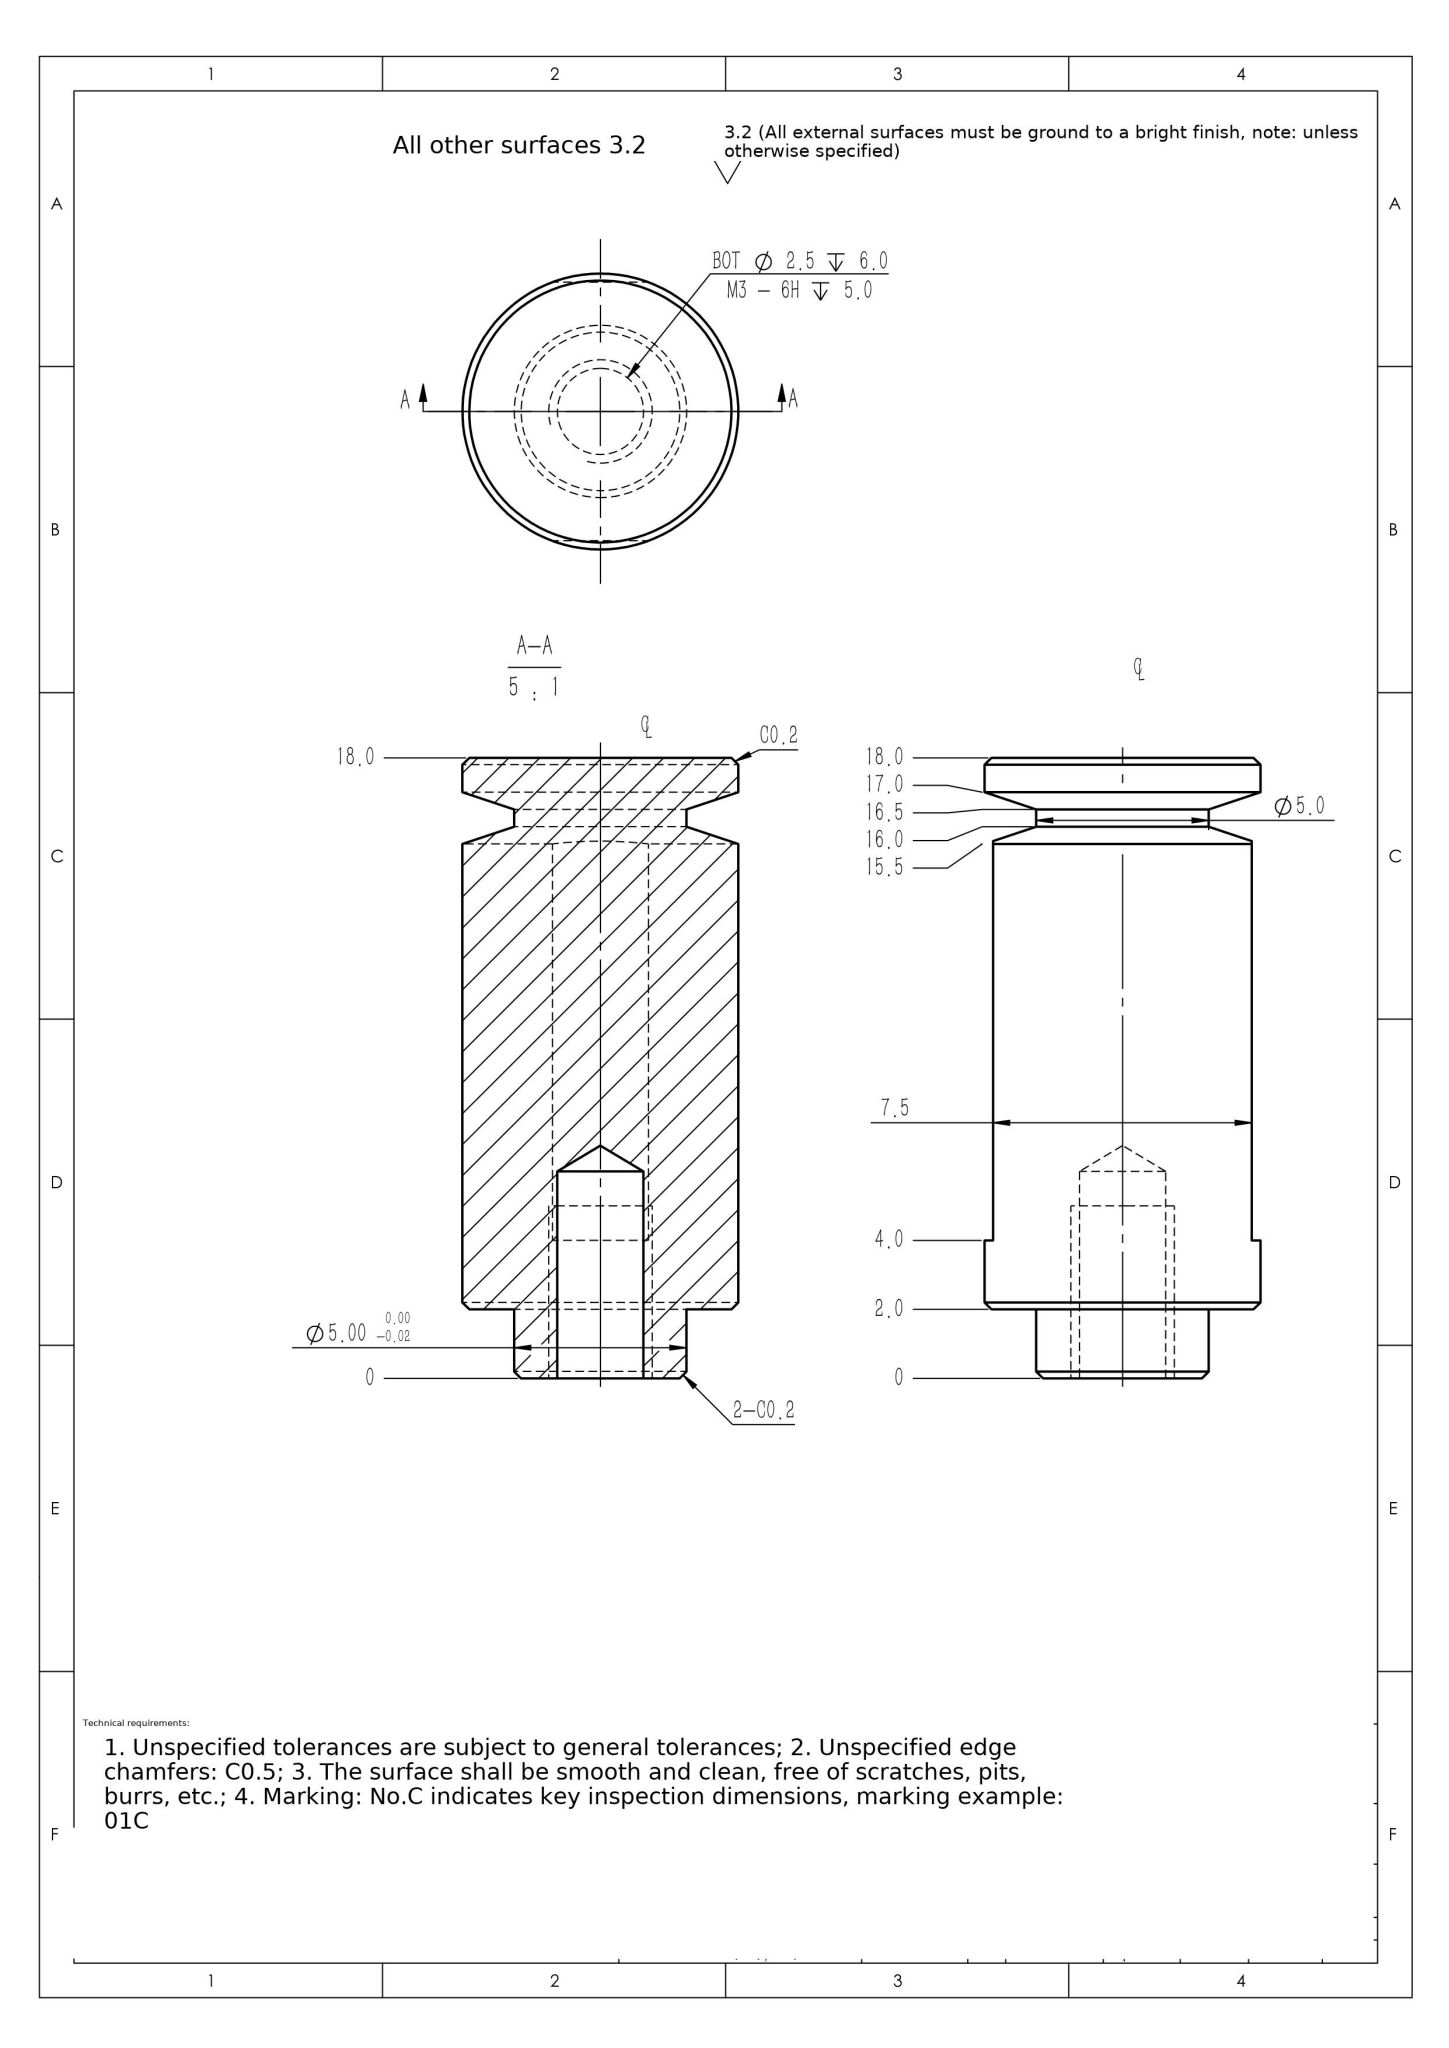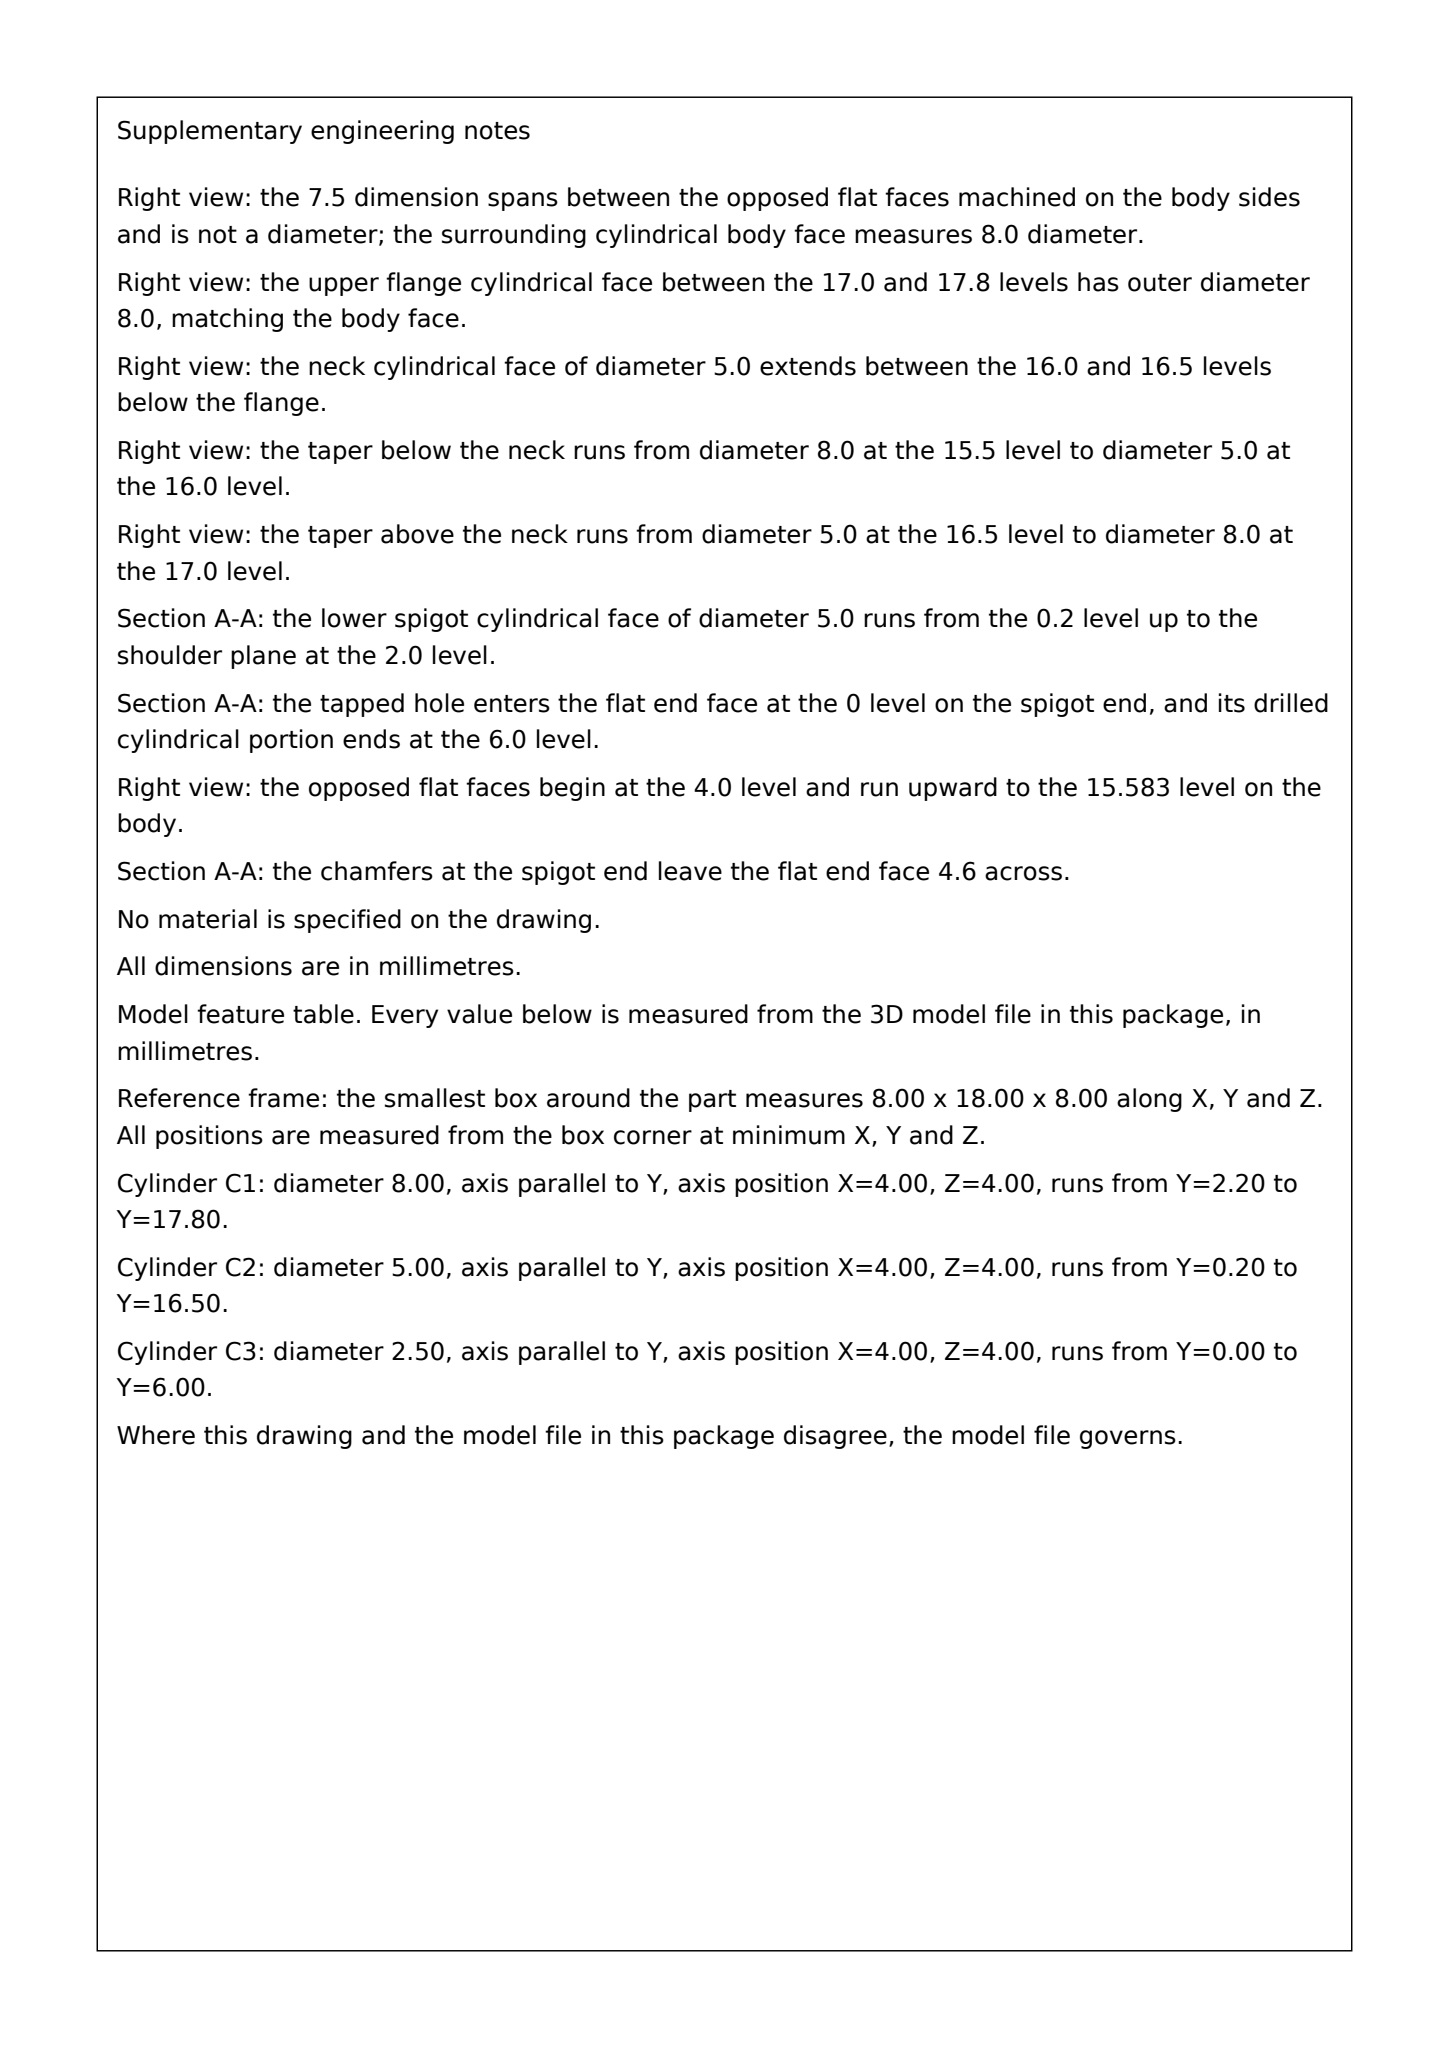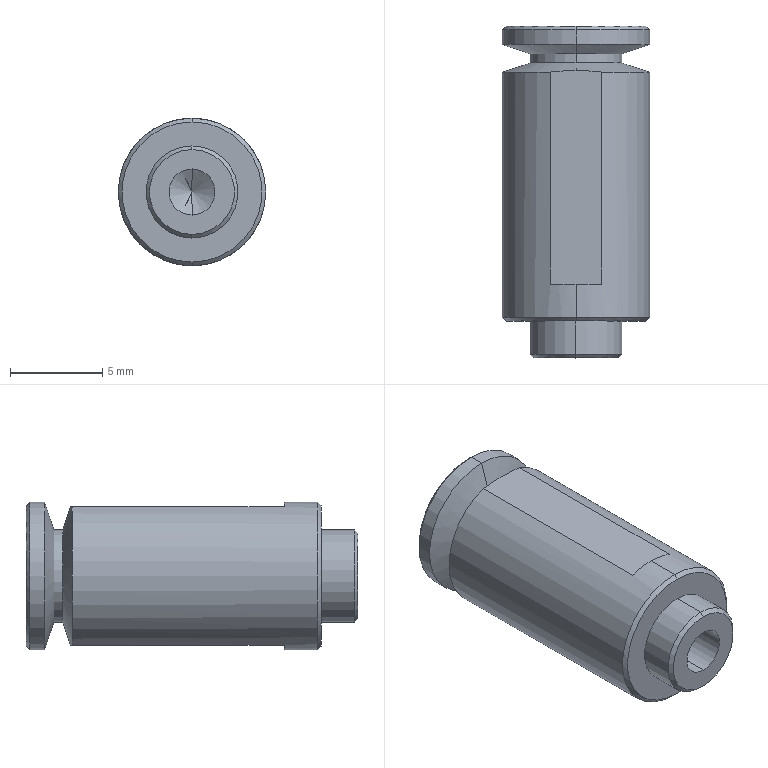Part | SolidWorks | mm | 1 solid | 29 faces | box 8 x 18 x 8 mm | volume 769 mm3 | cone 12 | cylinder 10 | plane 7 | commonest cylinder face diameters 5 x4 8 x4 2.5 x2
Drawing notes:
Ø8.0 BODY & HEAD OD (TYP, SEC A-A) | from the solid: cylinders dia 8.0, axis y, lengths 13.3 and 0.8, pos (4.0,4.0)
C0.2 AT Ø8.0 TO Ø5.00 BOSS SHOULDER, 2.0 FROM BOTTOM | from the solid: axis plane y=2.0 step from Ø8.0 body to Ø5.0 boss; chamfer ref dia 8.0 / 5.0
build123d program:
from build123d import *

# Parameters (mm, degrees)
SKETCH1_R             = 4
BOSS_EXTRUDE1_DEPTH   = 18
M3_TAPPED_HOLE1_D     = 2.5
M3_TAPPED_HOLE1_DEPTH = 6
M3_TAPPED_HOLE1_TIP   = 0.7511
CHAMFER1_SIZE         = 0.2
SKETCH6_W             = 1.126
SKETCH6_H             = 12
SKETCH6_W_2           = 1.355
CUT_EXTRUDE1_DEPTH    = 5
SKETCH9_R             = 4
SKETCH9_R_2           = 2.5
CUT_EXTRUDE2_DEPTH    = 2
CHAMFER2_SIZE         = 0.2


with BuildPart() as part:
    # Sketch1 → Boss-Extrude1 (new body)
    with BuildSketch(Plane(origin=(0, 0, 0), x_dir=(1, 0, 0), z_dir=(0, 1, 0))):
        with Locations(Location((0, 0, 0), (0, 0, 270))):
            Circle(SKETCH1_R)
    extrude(amount=BOSS_EXTRUDE1_DEPTH)

    # M3 Tapped Hole1
    with Locations(Plane(origin=(0, 0, 0), x_dir=(-1, 0, 0), z_dir=(0, -1, 0))):
        with Locations((0, 0)):
            Hole(M3_TAPPED_HOLE1_D / 2, depth=M3_TAPPED_HOLE1_DEPTH)
            with Locations((0, 0, -(M3_TAPPED_HOLE1_DEPTH + M3_TAPPED_HOLE1_TIP / 2))):  # 118° drill point
                Cone(0, M3_TAPPED_HOLE1_D / 2, M3_TAPPED_HOLE1_TIP, mode=Mode.SUBTRACT)

    # Chamfer1
    chamfer1_edges = [part.edges().sort_by_distance(p)[0] for p in [
        (0, 18, -4),
    ]]
    chamfer(chamfer1_edges, length=CHAMFER1_SIZE)

    # Sketch6 → Cut-Extrude1 (cut, symmetric)
    with BuildSketch(Plane(origin=(0, 0, 0), x_dir=(0, 0, -1), z_dir=(1, 0, 0))):
        with Locations((-4.313, 10)):
            Rectangle(SKETCH6_W, SKETCH6_H)
        with Locations((4.427, 10)):
            Rectangle(SKETCH6_W_2, SKETCH6_H)
    extrude(amount=CUT_EXTRUDE1_DEPTH, both=True, mode=Mode.SUBTRACT)

    # Sketch8 → Cut-Revolve1 (revolve, cut)
    with BuildSketch(Plane.XY, mode=Mode.PRIVATE) as cut_revolve1_sk:
        Polygon((-4, 17), (-2.5, 16.5), (-2.5, 16), (-4, 15.5), align=None)
    revolve(cut_revolve1_sk.sketch.rotate(Axis((0, 18, 0), (0, -1, 0)), 69.636), axis=Axis((0, 18, 0), (0, -1, 0)), mode=Mode.SUBTRACT)

    # Sketch9 → Cut-Extrude2 (cut)
    with BuildSketch(Plane.XZ):
        with Locations(Location((0, 0, 0), (0, 0, 270))):
            Circle(SKETCH9_R)
        with Locations(Location((0, 0, 0), (0, 0, 90))):
            Circle(SKETCH9_R_2, mode=Mode.SUBTRACT)
    extrude(amount=-CUT_EXTRUDE2_DEPTH, mode=Mode.SUBTRACT)

    # Chamfer2
    chamfer2_edges = [part.edges().sort_by_distance(p)[0] for p in [
        (0, 2, -4),
        (0, 0, -2.5),
    ]]
    chamfer(chamfer2_edges, length=CHAMFER2_SIZE)


solid = part.part
STEP:
#1=CARTESIAN_POINT('',(-0.,0.,-2.3));
#2=VERTEX_POINT('',#1);
#3=CARTESIAN_POINT('',(-0.,0.,2.3));
#4=VERTEX_POINT('',#3);
#5=CARTESIAN_POINT('',(-0.,0.,0.));
#6=DIRECTION('',(0.,-1.,0.));
#7=DIRECTION('',(0.,0.,1.));
#8=AXIS2_PLACEMENT_3D('',#5,#6,#7);
#9=CIRCLE('',#8,2.3);
#10=EDGE_CURVE('',#2,#4,#9,.T.);
#11=ORIENTED_EDGE('',*,*,#10,.F.);
#12=CARTESIAN_POINT('',(-0.,0.2,-2.5));
#13=VERTEX_POINT('',#12);
#14=CARTESIAN_POINT('',(-0.,0.,-2.3));
#15=DIRECTION('',(0.,0.7071,-0.7071));
#16=VECTOR('',#15,1000.);
#17=LINE('',#14,#16);
#18=EDGE_CURVE('',#2,#13,#17,.T.);
#19=ORIENTED_EDGE('',*,*,#18,.T.);
#20=CARTESIAN_POINT('',(-0.,0.2,2.5));
#21=VERTEX_POINT('',#20);
#22=CARTESIAN_POINT('',(-0.,0.2,0.));
#23=DIRECTION('',(0.,1.,0.));
#24=DIRECTION('',(0.,0.,1.));
#25=AXIS2_PLACEMENT_3D('',#22,#23,#24);
#26=CIRCLE('',#25,2.5);
#27=EDGE_CURVE('',#21,#13,#26,.T.);
#28=ORIENTED_EDGE('',*,*,#27,.F.);
#29=CARTESIAN_POINT('',(-0.,0.,2.3));
#30=DIRECTION('',(0.,0.7071,0.7071));
#31=VECTOR('',#30,1000.);
#32=LINE('',#29,#31);
#33=EDGE_CURVE('',#4,#21,#32,.T.);
#34=ORIENTED_EDGE('',*,*,#33,.F.);
#35=EDGE_LOOP('',(#11,#19,#28,#34));
#36=FACE_OUTER_BOUND('',#35,.T.);
#37=CARTESIAN_POINT('',(-0.,0.,0.));
#38=DIRECTION('',(0.,1.,0.));
#39=DIRECTION('',(0.,0.,1.));
#40=AXIS2_PLACEMENT_3D('',#37,#38,#39);
#41=CONICAL_SURFACE('',#40,2.3,0.7854);
#42=ADVANCED_FACE('',(#36),#41,.T.);
#43=CARTESIAN_POINT('',(0.,2.,-3.8));
#44=VERTEX_POINT('',#43);
#45=CARTESIAN_POINT('',(0.,2.,3.8));
#46=VERTEX_POINT('',#45);
#47=CARTESIAN_POINT('',(0.,2.,0.));
#48=DIRECTION('',(0.,-1.,0.));
#49=DIRECTION('',(0.,0.,-1.));
#50=AXIS2_PLACEMENT_3D('',#47,#48,#49);
#51=CIRCLE('',#50,3.8);
#52=EDGE_CURVE('',#44,#46,#51,.T.);
#53=ORIENTED_EDGE('',*,*,#52,.F.);
#54=CARTESIAN_POINT('',(0.,2.2,-4.));
#55=VERTEX_POINT('',#54);
#56=CARTESIAN_POINT('',(0.,2.,-3.8));
#57=DIRECTION('',(0.,0.7071,-0.7071));
#58=VECTOR('',#57,1000.);
#59=LINE('',#56,#58);
#60=EDGE_CURVE('',#44,#55,#59,.T.);
#61=ORIENTED_EDGE('',*,*,#60,.T.);
#62=CARTESIAN_POINT('',(0.,2.2,4.));
#63=VERTEX_POINT('',#62);
#64=CARTESIAN_POINT('',(0.,2.2,0.));
#65=DIRECTION('',(0.,1.,0.));
#66=DIRECTION('',(0.,0.,-1.));
#67=AXIS2_PLACEMENT_3D('',#64,#65,#66);
#68=CIRCLE('',#67,4.);
#69=EDGE_CURVE('',#63,#55,#68,.T.);
#70=ORIENTED_EDGE('',*,*,#69,.F.);
#71=CARTESIAN_POINT('',(0.,2.,3.8));
#72=DIRECTION('',(0.,0.7071,0.7071));
#73=VECTOR('',#72,1000.);
#74=LINE('',#71,#73);
#75=EDGE_CURVE('',#46,#63,#74,.T.);
#76=ORIENTED_EDGE('',*,*,#75,.F.);
#77=EDGE_LOOP('',(#53,#61,#70,#76));
#78=FACE_OUTER_BOUND('',#77,.T.);
#79=CARTESIAN_POINT('',(0.,2.,0.));
#80=DIRECTION('',(0.,1.,0.));
#81=DIRECTION('',(0.,0.,1.));
#82=AXIS2_PLACEMENT_3D('',#79,#80,#81);
#83=CONICAL_SURFACE('',#82,3.8,0.7854);
#84=ADVANCED_FACE('',(#78),#83,.T.);
#85=CARTESIAN_POINT('',(0.,6.,1.25));
#86=VERTEX_POINT('',#85);
#87=CARTESIAN_POINT('',(0.,6.,-1.25));
#88=VERTEX_POINT('',#87);
#89=CARTESIAN_POINT('',(0.,6.,0.));
#90=DIRECTION('',(0.,-1.,0.));
#91=DIRECTION('',(0.,0.,-1.));
#92=AXIS2_PLACEMENT_3D('',#89,#90,#91);
#93=CIRCLE('',#92,1.25);
#94=EDGE_CURVE('',#86,#88,#93,.T.);
#95=ORIENTED_EDGE('',*,*,#94,.F.);
#96=CARTESIAN_POINT('',(0.,-0.,1.25));
#97=VERTEX_POINT('',#96);
#98=CARTESIAN_POINT('',(0.,0.,1.25));
#99=DIRECTION('',(0.,-1.,0.));
#100=VECTOR('',#99,1000.);
#101=LINE('',#98,#100);
#102=EDGE_CURVE('',#86,#97,#101,.T.);
#103=ORIENTED_EDGE('',*,*,#102,.T.);
#104=CARTESIAN_POINT('',(0.,-0.,-1.25));
#105=VERTEX_POINT('',#104);
#106=CARTESIAN_POINT('',(0.,-0.,0.));
#107=DIRECTION('',(0.,-1.,0.));
#108=DIRECTION('',(0.,0.,-1.));
#109=AXIS2_PLACEMENT_3D('',#106,#107,#108);
#110=CIRCLE('',#109,1.25);
#111=EDGE_CURVE('',#97,#105,#110,.T.);
#112=ORIENTED_EDGE('',*,*,#111,.T.);
#113=CARTESIAN_POINT('',(0.,0.,-1.25));
#114=DIRECTION('',(0.,-1.,0.));
#115=VECTOR('',#114,1000.);
#116=LINE('',#113,#115);
#117=EDGE_CURVE('',#88,#105,#116,.T.);
#118=ORIENTED_EDGE('',*,*,#117,.F.);
#119=EDGE_LOOP('',(#95,#103,#112,#118));
#120=FACE_OUTER_BOUND('',#119,.T.);
#121=CARTESIAN_POINT('',(0.,0.,0.));
#122=DIRECTION('',(0.,-1.,0.));
#123=DIRECTION('',(0.,0.,-1.));
#124=AXIS2_PLACEMENT_3D('',#121,#122,#123);
#125=CYLINDRICAL_SURFACE('',#124,1.25);
#126=ADVANCED_FACE('',(#120),#125,.F.);
#127=CARTESIAN_POINT('',(-0.,6.751,0.));
#128=VERTEX_POINT('',#127);
#129=CARTESIAN_POINT('',(0.,6.,-1.25));
#130=DIRECTION('',(0.,-0.515,-0.8572));
#131=VECTOR('',#130,1000.);
#132=LINE('',#129,#131);
#133=EDGE_CURVE('',#128,#88,#132,.T.);
#134=ORIENTED_EDGE('',*,*,#133,.F.);
#135=CARTESIAN_POINT('',(0.,6.,1.25));
#136=DIRECTION('',(0.,-0.515,0.8572));
#137=VECTOR('',#136,1000.);
#138=LINE('',#135,#137);
#139=EDGE_CURVE('',#128,#86,#138,.T.);
#140=ORIENTED_EDGE('',*,*,#139,.T.);
#141=ORIENTED_EDGE('',*,*,#94,.T.);
#142=EDGE_LOOP('',(#134,#140,#141));
#143=FACE_OUTER_BOUND('',#142,.T.);
#144=CARTESIAN_POINT('',(0.,6.,0.));
#145=DIRECTION('',(0.,-1.,0.));
#146=DIRECTION('',(0.,0.,-1.));
#147=AXIS2_PLACEMENT_3D('',#144,#145,#146);
#148=CONICAL_SURFACE('',#147,1.25,1.03);
#149=ADVANCED_FACE('',(#143),#148,.F.);
#150=CARTESIAN_POINT('',(-0.,2.,-2.5));
#151=VERTEX_POINT('',#150);
#152=CARTESIAN_POINT('',(-0.,2.,2.5));
#153=VERTEX_POINT('',#152);
#154=CARTESIAN_POINT('',(-0.,2.,0.));
#155=DIRECTION('',(0.,-1.,0.));
#156=DIRECTION('',(0.,0.,-1.));
#157=AXIS2_PLACEMENT_3D('',#154,#155,#156);
#158=CIRCLE('',#157,2.5);
#159=EDGE_CURVE('',#151,#153,#158,.T.);
#160=ORIENTED_EDGE('',*,*,#159,.T.);
#161=CARTESIAN_POINT('',(-0.,2.,2.5));
#162=DIRECTION('',(0.,-1.,0.));
#163=VECTOR('',#162,1000.);
#164=LINE('',#161,#163);
#165=EDGE_CURVE('',#153,#21,#164,.T.);
#166=ORIENTED_EDGE('',*,*,#165,.T.);
#167=ORIENTED_EDGE('',*,*,#27,.T.);
#168=CARTESIAN_POINT('',(-0.,2.,-2.5));
#169=DIRECTION('',(0.,-1.,0.));
#170=VECTOR('',#169,1000.);
#171=LINE('',#168,#170);
#172=EDGE_CURVE('',#151,#13,#171,.T.);
#173=ORIENTED_EDGE('',*,*,#172,.F.);
#174=EDGE_LOOP('',(#160,#166,#167,#173));
#175=FACE_OUTER_BOUND('',#174,.T.);
#176=CARTESIAN_POINT('',(-0.,2.,0.));
#177=DIRECTION('',(0.,-1.,0.));
#178=DIRECTION('',(0.,0.,-1.));
#179=AXIS2_PLACEMENT_3D('',#176,#177,#178);
#180=CYLINDRICAL_SURFACE('',#179,2.5);
#181=ADVANCED_FACE('',(#175),#180,.T.);
#182=CARTESIAN_POINT('',(0.,17.8,-4.));
#183=VERTEX_POINT('',#182);
#184=CARTESIAN_POINT('',(0.,17.8,4.));
#185=VERTEX_POINT('',#184);
#186=CARTESIAN_POINT('',(0.,17.8,0.));
#187=DIRECTION('',(0.,-1.,0.));
#188=DIRECTION('',(0.,0.,1.));
#189=AXIS2_PLACEMENT_3D('',#186,#187,#188);
#190=CIRCLE('',#189,4.);
#191=EDGE_CURVE('',#183,#185,#190,.T.);
#192=ORIENTED_EDGE('',*,*,#191,.T.);
#193=CARTESIAN_POINT('',(0.,17.,4.));
#194=VERTEX_POINT('',#193);
#195=CARTESIAN_POINT('',(0.,18.,4.));
#196=DIRECTION('',(0.,-1.,0.));
#197=VECTOR('',#196,1000.);
#198=LINE('',#195,#197);
#199=EDGE_CURVE('',#185,#194,#198,.T.);
#200=ORIENTED_EDGE('',*,*,#199,.T.);
#201=CARTESIAN_POINT('',(0.,17.,-4.));
#202=VERTEX_POINT('',#201);
#203=CARTESIAN_POINT('',(0.,17.,0.));
#204=DIRECTION('',(0.,1.,0.));
#205=DIRECTION('',(0.,0.,1.));
#206=AXIS2_PLACEMENT_3D('',#203,#204,#205);
#207=CIRCLE('',#206,4.);
#208=EDGE_CURVE('',#194,#202,#207,.T.);
#209=ORIENTED_EDGE('',*,*,#208,.T.);
#210=CARTESIAN_POINT('',(0.,18.,-4.));
#211=DIRECTION('',(0.,-1.,0.));
#212=VECTOR('',#211,1000.);
#213=LINE('',#210,#212);
#214=EDGE_CURVE('',#183,#202,#213,.T.);
#215=ORIENTED_EDGE('',*,*,#214,.F.);
#216=EDGE_LOOP('',(#192,#200,#209,#215));
#217=FACE_OUTER_BOUND('',#216,.T.);
#218=CARTESIAN_POINT('',(0.,18.,0.));
#219=DIRECTION('',(0.,-1.,0.));
#220=DIRECTION('',(0.,0.,-1.));
#221=AXIS2_PLACEMENT_3D('',#218,#219,#220);
#222=CYLINDRICAL_SURFACE('',#221,4.);
#223=ADVANCED_FACE('',(#217),#222,.T.);
#224=CARTESIAN_POINT('',(0.,18.,3.8));
#225=VERTEX_POINT('',#224);
#226=CARTESIAN_POINT('',(0.,18.,-3.8));
#227=VERTEX_POINT('',#226);
#228=CARTESIAN_POINT('',(0.,18.,0.));
#229=DIRECTION('',(0.,1.,0.));
#230=DIRECTION('',(0.,0.,1.));
#231=AXIS2_PLACEMENT_3D('',#228,#229,#230);
#232=CIRCLE('',#231,3.8);
#233=EDGE_CURVE('',#225,#227,#232,.T.);
#234=ORIENTED_EDGE('',*,*,#233,.F.);
#235=CARTESIAN_POINT('',(0.,18.,3.8));
#236=DIRECTION('',(0.,-0.7071,0.7071));
#237=VECTOR('',#236,1000.);
#238=LINE('',#235,#237);
#239=EDGE_CURVE('',#225,#185,#238,.T.);
#240=ORIENTED_EDGE('',*,*,#239,.T.);
#241=ORIENTED_EDGE('',*,*,#191,.F.);
#242=CARTESIAN_POINT('',(0.,18.,-3.8));
#243=DIRECTION('',(0.,-0.7071,-0.7071));
#244=VECTOR('',#243,1000.);
#245=LINE('',#242,#244);
#246=EDGE_CURVE('',#227,#183,#245,.T.);
#247=ORIENTED_EDGE('',*,*,#246,.F.);
#248=EDGE_LOOP('',(#234,#240,#241,#247));
#249=FACE_OUTER_BOUND('',#248,.T.);
#250=CARTESIAN_POINT('',(0.,18.,0.));
#251=DIRECTION('',(0.,-1.,0.));
#252=DIRECTION('',(0.,0.,-1.));
#253=AXIS2_PLACEMENT_3D('',#250,#251,#252);
#254=CONICAL_SURFACE('',#253,3.8,0.7854);
#255=ADVANCED_FACE('',(#249),#254,.T.);
#256=CARTESIAN_POINT('',(0.,16.,2.5));
#257=VERTEX_POINT('',#256);
#258=CARTESIAN_POINT('',(0.,16.,-2.5));
#259=VERTEX_POINT('',#258);
#260=CARTESIAN_POINT('',(0.,16.,0.));
#261=DIRECTION('',(0.,1.,0.));
#262=DIRECTION('',(0.,0.,1.));
#263=AXIS2_PLACEMENT_3D('',#260,#261,#262);
#264=CIRCLE('',#263,2.5);
#265=EDGE_CURVE('',#257,#259,#264,.T.);
#266=ORIENTED_EDGE('',*,*,#265,.T.);
#267=CARTESIAN_POINT('',(0.,16.5,-2.5));
#268=VERTEX_POINT('',#267);
#269=CARTESIAN_POINT('',(0.,18.,-2.5));
#270=DIRECTION('',(0.,1.,0.));
#271=VECTOR('',#270,1000.);
#272=LINE('',#269,#271);
#273=EDGE_CURVE('',#259,#268,#272,.T.);
#274=ORIENTED_EDGE('',*,*,#273,.T.);
#275=CARTESIAN_POINT('',(0.,16.5,2.5));
#276=VERTEX_POINT('',#275);
#277=CARTESIAN_POINT('',(0.,16.5,0.));
#278=DIRECTION('',(0.,1.,0.));
#279=DIRECTION('',(0.,0.,1.));
#280=AXIS2_PLACEMENT_3D('',#277,#278,#279);
#281=CIRCLE('',#280,2.5);
#282=EDGE_CURVE('',#276,#268,#281,.T.);
#283=ORIENTED_EDGE('',*,*,#282,.F.);
#284=CARTESIAN_POINT('',(0.,18.,2.5));
#285=DIRECTION('',(0.,1.,0.));
#286=VECTOR('',#285,1000.);
#287=LINE('',#284,#286);
#288=EDGE_CURVE('',#257,#276,#287,.T.);
#289=ORIENTED_EDGE('',*,*,#288,.F.);
#290=EDGE_LOOP('',(#266,#274,#283,#289));
#291=FACE_OUTER_BOUND('',#290,.T.);
#292=CARTESIAN_POINT('',(0.,18.,0.));
#293=DIRECTION('',(0.,1.,0.));
#294=DIRECTION('',(0.,0.,1.));
#295=AXIS2_PLACEMENT_3D('',#292,#293,#294);
#296=CYLINDRICAL_SURFACE('',#295,2.5);
#297=ADVANCED_FACE('',(#291),#296,.T.);
#298=ORIENTED_EDGE('',*,*,#282,.T.);
#299=CARTESIAN_POINT('',(0.,16.5,-2.5));
#300=DIRECTION('',(0.,0.3162,-0.9487));
#301=VECTOR('',#300,1000.);
#302=LINE('',#299,#301);
#303=EDGE_CURVE('',#268,#202,#302,.T.);
#304=ORIENTED_EDGE('',*,*,#303,.T.);
#305=ORIENTED_EDGE('',*,*,#208,.F.);
#306=CARTESIAN_POINT('',(0.,16.5,2.5));
#307=DIRECTION('',(0.,0.3162,0.9487));
#308=VECTOR('',#307,1000.);
#309=LINE('',#306,#308);
#310=EDGE_CURVE('',#276,#194,#309,.T.);
#311=ORIENTED_EDGE('',*,*,#310,.F.);
#312=EDGE_LOOP('',(#298,#304,#305,#311));
#313=FACE_OUTER_BOUND('',#312,.T.);
#314=CARTESIAN_POINT('',(0.,16.5,0.));
#315=DIRECTION('',(0.,1.,0.));
#316=DIRECTION('',(0.,0.,1.));
#317=AXIS2_PLACEMENT_3D('',#314,#315,#316);
#318=CONICAL_SURFACE('',#317,2.5,1.249);
#319=ADVANCED_FACE('',(#313),#318,.T.);
#320=ORIENTED_EDGE('',*,*,#265,.F.);
#321=CARTESIAN_POINT('',(0.,15.583,3.75));
#322=VERTEX_POINT('',#321);
#323=CARTESIAN_POINT('',(0.,15.5,4.));
#324=DIRECTION('',(0.,-0.3162,0.9487));
#325=VECTOR('',#324,1000.);
#326=LINE('',#323,#325);
#327=EDGE_CURVE('',#257,#322,#326,.T.);
#328=ORIENTED_EDGE('',*,*,#327,.T.);
#329=CARTESIAN_POINT('',(1.392,15.5,3.75));
#330=VERTEX_POINT('',#329);
#331=CARTESIAN_POINT('',(1.392,15.5,3.75));
#332=CARTESIAN_POINT('',(0.9298,15.554,3.75));
#333=CARTESIAN_POINT('',(0.466,15.583,3.75));
#334=CARTESIAN_POINT('',(0.,15.583,3.75));
#335=B_SPLINE_CURVE_WITH_KNOTS('',3,(#331,#332,#333,#334),.UNSPECIFIED.,.F.,.F.,(4,4),(0.001505,0.002899),.UNSPECIFIED.);
#336=EDGE_CURVE('',#330,#322,#335,.T.);
#337=ORIENTED_EDGE('',*,*,#336,.F.);
#338=CARTESIAN_POINT('',(1.392,15.5,-3.75));
#339=VERTEX_POINT('',#338);
#340=CARTESIAN_POINT('',(0.,15.5,0.));
#341=DIRECTION('',(0.,1.,0.));
#342=DIRECTION('',(0.,0.,1.));
#343=AXIS2_PLACEMENT_3D('',#340,#341,#342);
#344=CIRCLE('',#343,4.);
#345=EDGE_CURVE('',#330,#339,#344,.T.);
#346=ORIENTED_EDGE('',*,*,#345,.T.);
#347=CARTESIAN_POINT('',(0.,15.583,-3.75));
#348=VERTEX_POINT('',#347);
#349=CARTESIAN_POINT('',(0.,15.583,-3.75));
#350=CARTESIAN_POINT('',(0.466,15.583,-3.75));
#351=CARTESIAN_POINT('',(0.9298,15.554,-3.75));
#352=CARTESIAN_POINT('',(1.392,15.5,-3.75));
#353=B_SPLINE_CURVE_WITH_KNOTS('',3,(#349,#350,#351,#352),.UNSPECIFIED.,.F.,.F.,(4,4),(0.005039,0.006443),.UNSPECIFIED.);
#354=EDGE_CURVE('',#348,#339,#353,.T.);
#355=ORIENTED_EDGE('',*,*,#354,.F.);
#356=CARTESIAN_POINT('',(0.,15.5,-4.));
#357=DIRECTION('',(0.,-0.3162,-0.9487));
#358=VECTOR('',#357,1000.);
#359=LINE('',#356,#358);
#360=EDGE_CURVE('',#259,#348,#359,.T.);
#361=ORIENTED_EDGE('',*,*,#360,.F.);
#362=EDGE_LOOP('',(#320,#328,#337,#346,#355,#361));
#363=FACE_OUTER_BOUND('',#362,.T.);
#364=CARTESIAN_POINT('',(0.,15.5,0.));
#365=DIRECTION('',(0.,-1.,0.));
#366=DIRECTION('',(0.,0.,-1.));
#367=AXIS2_PLACEMENT_3D('',#364,#365,#366);
#368=CONICAL_SURFACE('',#367,4.,1.249);
#369=ADVANCED_FACE('',(#363),#368,.T.);
#370=CARTESIAN_POINT('',(1.392,4.,3.75));
#371=VERTEX_POINT('',#370);
#372=CARTESIAN_POINT('',(0.,4.,4.));
#373=VERTEX_POINT('',#372);
#374=CARTESIAN_POINT('',(0.,4.,0.));
#375=DIRECTION('',(0.,-1.,0.));
#376=DIRECTION('',(0.,0.,-1.));
#377=AXIS2_PLACEMENT_3D('',#374,#375,#376);
#378=CIRCLE('',#377,4.);
#379=EDGE_CURVE('',#371,#373,#378,.T.);
#380=ORIENTED_EDGE('',*,*,#379,.T.);
#381=CARTESIAN_POINT('',(0.,18.,4.));
#382=DIRECTION('',(0.,-1.,0.));
#383=VECTOR('',#382,1000.);
#384=LINE('',#381,#383);
#385=EDGE_CURVE('',#373,#63,#384,.T.);
#386=ORIENTED_EDGE('',*,*,#385,.T.);
#387=ORIENTED_EDGE('',*,*,#69,.T.);
#388=CARTESIAN_POINT('',(0.,4.,-4.));
#389=VERTEX_POINT('',#388);
#390=CARTESIAN_POINT('',(0.,18.,-4.));
#391=DIRECTION('',(0.,-1.,0.));
#392=VECTOR('',#391,1000.);
#393=LINE('',#390,#392);
#394=EDGE_CURVE('',#389,#55,#393,.T.);
#395=ORIENTED_EDGE('',*,*,#394,.F.);
#396=CARTESIAN_POINT('',(1.392,4.,-3.75));
#397=VERTEX_POINT('',#396);
#398=CARTESIAN_POINT('',(0.,4.,0.));
#399=DIRECTION('',(0.,-1.,0.));
#400=DIRECTION('',(0.,0.,-1.));
#401=AXIS2_PLACEMENT_3D('',#398,#399,#400);
#402=CIRCLE('',#401,4.);
#403=EDGE_CURVE('',#389,#397,#402,.T.);
#404=ORIENTED_EDGE('',*,*,#403,.T.);
#405=CARTESIAN_POINT('',(1.392,18.,-3.75));
#406=DIRECTION('',(0.,1.,0.));
#407=VECTOR('',#406,1000.);
#408=LINE('',#405,#407);
#409=EDGE_CURVE('',#397,#339,#408,.T.);
#410=ORIENTED_EDGE('',*,*,#409,.T.);
#411=ORIENTED_EDGE('',*,*,#345,.F.);
#412=CARTESIAN_POINT('',(1.392,18.,3.75));
#413=DIRECTION('',(0.,-1.,0.));
#414=VECTOR('',#413,1000.);
#415=LINE('',#412,#414);
#416=EDGE_CURVE('',#330,#371,#415,.T.);
#417=ORIENTED_EDGE('',*,*,#416,.T.);
#418=EDGE_LOOP('',(#380,#386,#387,#395,#404,#410,#411,#417));
#419=FACE_OUTER_BOUND('',#418,.T.);
#420=CARTESIAN_POINT('',(0.,18.,0.));
#421=DIRECTION('',(0.,-1.,0.));
#422=DIRECTION('',(0.,0.,-1.));
#423=AXIS2_PLACEMENT_3D('',#420,#421,#422);
#424=CYLINDRICAL_SURFACE('',#423,4.);
#425=ADVANCED_FACE('',(#419),#424,.T.);
#426=ORIENTED_EDGE('',*,*,#385,.F.);
#427=CARTESIAN_POINT('',(-1.392,4.,3.75));
#428=VERTEX_POINT('',#427);
#429=CARTESIAN_POINT('',(0.,4.,0.));
#430=DIRECTION('',(0.,-1.,0.));
#431=DIRECTION('',(0.,0.,-1.));
#432=AXIS2_PLACEMENT_3D('',#429,#430,#431);
#433=CIRCLE('',#432,4.);
#434=EDGE_CURVE('',#373,#428,#433,.T.);
#435=ORIENTED_EDGE('',*,*,#434,.T.);
#436=CARTESIAN_POINT('',(-1.392,15.5,3.75));
#437=VERTEX_POINT('',#436);
#438=CARTESIAN_POINT('',(-1.392,18.,3.75));
#439=DIRECTION('',(0.,1.,0.));
#440=VECTOR('',#439,1000.);
#441=LINE('',#438,#440);
#442=EDGE_CURVE('',#428,#437,#441,.T.);
#443=ORIENTED_EDGE('',*,*,#442,.T.);
#444=CARTESIAN_POINT('',(-1.392,15.5,-3.75));
#445=VERTEX_POINT('',#444);
#446=CARTESIAN_POINT('',(0.,15.5,0.));
#447=DIRECTION('',(0.,1.,0.));
#448=DIRECTION('',(0.,0.,1.));
#449=AXIS2_PLACEMENT_3D('',#446,#447,#448);
#450=CIRCLE('',#449,4.);
#451=EDGE_CURVE('',#445,#437,#450,.T.);
#452=ORIENTED_EDGE('',*,*,#451,.F.);
#453=CARTESIAN_POINT('',(-1.392,4.,-3.75));
#454=VERTEX_POINT('',#453);
#455=CARTESIAN_POINT('',(-1.392,18.,-3.75));
#456=DIRECTION('',(0.,-1.,0.));
#457=VECTOR('',#456,1000.);
#458=LINE('',#455,#457);
#459=EDGE_CURVE('',#445,#454,#458,.T.);
#460=ORIENTED_EDGE('',*,*,#459,.T.);
#461=CARTESIAN_POINT('',(0.,4.,0.));
#462=DIRECTION('',(0.,-1.,0.));
#463=DIRECTION('',(0.,0.,-1.));
#464=AXIS2_PLACEMENT_3D('',#461,#462,#463);
#465=CIRCLE('',#464,4.);
#466=EDGE_CURVE('',#454,#389,#465,.T.);
#467=ORIENTED_EDGE('',*,*,#466,.T.);
#468=ORIENTED_EDGE('',*,*,#394,.T.);
#469=CARTESIAN_POINT('',(0.,2.2,0.));
#470=DIRECTION('',(0.,1.,0.));
#471=DIRECTION('',(0.,0.,-1.));
#472=AXIS2_PLACEMENT_3D('',#469,#470,#471);
#473=CIRCLE('',#472,4.);
#474=EDGE_CURVE('',#55,#63,#473,.T.);
#475=ORIENTED_EDGE('',*,*,#474,.T.);
#476=EDGE_LOOP('',(#426,#435,#443,#452,#460,#467,#468,#475));
#477=FACE_OUTER_BOUND('',#476,.T.);
#478=CARTESIAN_POINT('',(0.,18.,0.));
#479=DIRECTION('',(0.,-1.,0.));
#480=DIRECTION('',(0.,0.,-1.));
#481=AXIS2_PLACEMENT_3D('',#478,#479,#480);
#482=CYLINDRICAL_SURFACE('',#481,4.);
#483=ADVANCED_FACE('',(#477),#482,.T.);
#484=ORIENTED_EDGE('',*,*,#416,.F.);
#485=ORIENTED_EDGE('',*,*,#336,.T.);
#486=CARTESIAN_POINT('',(0.,15.583,3.75));
#487=CARTESIAN_POINT('',(-0.4624,15.583,3.75));
#488=CARTESIAN_POINT('',(-0.9291,15.554,3.75));
#489=CARTESIAN_POINT('',(-1.392,15.5,3.75));
#490=B_SPLINE_CURVE_WITH_KNOTS('',3,(#486,#487,#488,#489),.UNSPECIFIED.,.F.,.F.,(4,4),(0.002899,0.004283),.UNSPECIFIED.);
#491=EDGE_CURVE('',#322,#437,#490,.T.);
#492=ORIENTED_EDGE('',*,*,#491,.T.);
#493=ORIENTED_EDGE('',*,*,#442,.F.);
#494=CARTESIAN_POINT('',(-5.,4.,3.75));
#495=DIRECTION('',(1.,0.,0.));
#496=VECTOR('',#495,1000.);
#497=LINE('',#494,#496);
#498=EDGE_CURVE('',#428,#371,#497,.T.);
#499=ORIENTED_EDGE('',*,*,#498,.T.);
#500=EDGE_LOOP('',(#484,#485,#492,#493,#499));
#501=FACE_OUTER_BOUND('',#500,.T.);
#502=CARTESIAN_POINT('',(-5.,16.,3.75));
#503=DIRECTION('',(0.,-0.,-1.));
#504=DIRECTION('',(0.,1.,-0.));
#505=AXIS2_PLACEMENT_3D('',#502,#503,#504);
#506=PLANE('',#505);
#507=ADVANCED_FACE('',(#501),#506,.F.);
#508=ORIENTED_EDGE('',*,*,#498,.F.);
#509=ORIENTED_EDGE('',*,*,#434,.F.);
#510=ORIENTED_EDGE('',*,*,#379,.F.);
#511=EDGE_LOOP('',(#508,#509,#510));
#512=FACE_OUTER_BOUND('',#511,.T.);
#513=CARTESIAN_POINT('',(-5.,4.,4.876));
#514=DIRECTION('',(0.,-1.,0.));
#515=DIRECTION('',(0.,0.,-1.));
#516=AXIS2_PLACEMENT_3D('',#513,#514,#515);
#517=PLANE('',#516);
#518=ADVANCED_FACE('',(#512),#517,.F.);
#519=CARTESIAN_POINT('',(-5.,4.,-3.75));
#520=DIRECTION('',(1.,0.,0.));
#521=VECTOR('',#520,1000.);
#522=LINE('',#519,#521);
#523=EDGE_CURVE('',#454,#397,#522,.T.);
#524=ORIENTED_EDGE('',*,*,#523,.T.);
#525=ORIENTED_EDGE('',*,*,#403,.F.);
#526=ORIENTED_EDGE('',*,*,#466,.F.);
#527=EDGE_LOOP('',(#524,#525,#526));
#528=FACE_OUTER_BOUND('',#527,.T.);
#529=CARTESIAN_POINT('',(-5.,4.,-5.105));
#530=DIRECTION('',(0.,-1.,0.));
#531=DIRECTION('',(0.,0.,-1.));
#532=AXIS2_PLACEMENT_3D('',#529,#530,#531);
#533=PLANE('',#532);
#534=ADVANCED_FACE('',(#528),#533,.F.);
#535=ORIENTED_EDGE('',*,*,#459,.F.);
#536=CARTESIAN_POINT('',(-1.392,15.5,-3.75));
#537=CARTESIAN_POINT('',(-0.9291,15.554,-3.75));
#538=CARTESIAN_POINT('',(-0.4624,15.583,-3.75));
#539=CARTESIAN_POINT('',(0.,15.583,-3.75));
#540=B_SPLINE_CURVE_WITH_KNOTS('',3,(#536,#537,#538,#539),.UNSPECIFIED.,.F.,.F.,(4,4),(0.003646,0.005039),.UNSPECIFIED.);
#541=EDGE_CURVE('',#445,#348,#540,.T.);
#542=ORIENTED_EDGE('',*,*,#541,.T.);
#543=ORIENTED_EDGE('',*,*,#354,.T.);
#544=ORIENTED_EDGE('',*,*,#409,.F.);
#545=ORIENTED_EDGE('',*,*,#523,.F.);
#546=EDGE_LOOP('',(#535,#542,#543,#544,#545));
#547=FACE_OUTER_BOUND('',#546,.T.);
#548=CARTESIAN_POINT('',(-5.,16.,-3.75));
#549=DIRECTION('',(0.,-0.,1.));
#550=DIRECTION('',(0.,-1.,-0.));
#551=AXIS2_PLACEMENT_3D('',#548,#549,#550);
#552=PLANE('',#551);
#553=ADVANCED_FACE('',(#547),#552,.F.);
#554=ORIENTED_EDGE('',*,*,#327,.F.);
#555=CARTESIAN_POINT('',(0.,16.,0.));
#556=DIRECTION('',(0.,1.,0.));
#557=DIRECTION('',(0.,0.,1.));
#558=AXIS2_PLACEMENT_3D('',#555,#556,#557);
#559=CIRCLE('',#558,2.5);
#560=EDGE_CURVE('',#259,#257,#559,.T.);
#561=ORIENTED_EDGE('',*,*,#560,.F.);
#562=ORIENTED_EDGE('',*,*,#360,.T.);
#563=ORIENTED_EDGE('',*,*,#541,.F.);
#564=ORIENTED_EDGE('',*,*,#451,.T.);
#565=ORIENTED_EDGE('',*,*,#491,.F.);
#566=EDGE_LOOP('',(#554,#561,#562,#563,#564,#565));
#567=FACE_OUTER_BOUND('',#566,.T.);
#568=CARTESIAN_POINT('',(0.,15.5,0.));
#569=DIRECTION('',(0.,-1.,0.));
#570=DIRECTION('',(0.,0.,-1.));
#571=AXIS2_PLACEMENT_3D('',#568,#569,#570);
#572=CONICAL_SURFACE('',#571,4.,1.249);
#573=ADVANCED_FACE('',(#567),#572,.T.);
#574=ORIENTED_EDGE('',*,*,#303,.F.);
#575=CARTESIAN_POINT('',(0.,16.5,0.));
#576=DIRECTION('',(0.,1.,0.));
#577=DIRECTION('',(0.,0.,1.));
#578=AXIS2_PLACEMENT_3D('',#575,#576,#577);
#579=CIRCLE('',#578,2.5);
#580=EDGE_CURVE('',#268,#276,#579,.T.);
#581=ORIENTED_EDGE('',*,*,#580,.T.);
#582=ORIENTED_EDGE('',*,*,#310,.T.);
#583=CARTESIAN_POINT('',(0.,17.,0.));
#584=DIRECTION('',(0.,1.,0.));
#585=DIRECTION('',(0.,0.,1.));
#586=AXIS2_PLACEMENT_3D('',#583,#584,#585);
#587=CIRCLE('',#586,4.);
#588=EDGE_CURVE('',#202,#194,#587,.T.);
#589=ORIENTED_EDGE('',*,*,#588,.F.);
#590=EDGE_LOOP('',(#574,#581,#582,#589));
#591=FACE_OUTER_BOUND('',#590,.T.);
#592=CARTESIAN_POINT('',(0.,16.5,0.));
#593=DIRECTION('',(0.,1.,0.));
#594=DIRECTION('',(0.,0.,1.));
#595=AXIS2_PLACEMENT_3D('',#592,#593,#594);
#596=CONICAL_SURFACE('',#595,2.5,1.249);
#597=ADVANCED_FACE('',(#591),#596,.T.);
#598=ORIENTED_EDGE('',*,*,#273,.F.);
#599=ORIENTED_EDGE('',*,*,#560,.T.);
#600=ORIENTED_EDGE('',*,*,#288,.T.);
#601=ORIENTED_EDGE('',*,*,#580,.F.);
#602=EDGE_LOOP('',(#598,#599,#600,#601));
#603=FACE_OUTER_BOUND('',#602,.T.);
#604=CARTESIAN_POINT('',(0.,18.,0.));
#605=DIRECTION('',(0.,1.,0.));
#606=DIRECTION('',(0.,0.,1.));
#607=AXIS2_PLACEMENT_3D('',#604,#605,#606);
#608=CYLINDRICAL_SURFACE('',#607,2.5);
#609=ADVANCED_FACE('',(#603),#608,.T.);
#610=CARTESIAN_POINT('',(0.,18.,0.));
#611=DIRECTION('',(0.,1.,0.));
#612=DIRECTION('',(0.,0.,1.));
#613=AXIS2_PLACEMENT_3D('',#610,#611,#612);
#614=CIRCLE('',#613,3.8);
#615=EDGE_CURVE('',#227,#225,#614,.T.);
#616=ORIENTED_EDGE('',*,*,#615,.T.);
#617=ORIENTED_EDGE('',*,*,#233,.T.);
#618=EDGE_LOOP('',(#616,#617));
#619=FACE_OUTER_BOUND('',#618,.T.);
#620=CARTESIAN_POINT('',(0.,18.,0.));
#621=DIRECTION('',(0.,1.,0.));
#622=DIRECTION('',(0.,0.,1.));
#623=AXIS2_PLACEMENT_3D('',#620,#621,#622);
#624=PLANE('',#623);
#625=ADVANCED_FACE('',(#619),#624,.T.);
#626=ORIENTED_EDGE('',*,*,#239,.F.);
#627=ORIENTED_EDGE('',*,*,#615,.F.);
#628=ORIENTED_EDGE('',*,*,#246,.T.);
#629=CARTESIAN_POINT('',(0.,17.8,0.));
#630=DIRECTION('',(0.,-1.,0.));
#631=DIRECTION('',(0.,0.,1.));
#632=AXIS2_PLACEMENT_3D('',#629,#630,#631);
#633=CIRCLE('',#632,4.);
#634=EDGE_CURVE('',#185,#183,#633,.T.);
#635=ORIENTED_EDGE('',*,*,#634,.F.);
#636=EDGE_LOOP('',(#626,#627,#628,#635));
#637=FACE_OUTER_BOUND('',#636,.T.);
#638=CARTESIAN_POINT('',(0.,18.,0.));
#639=DIRECTION('',(0.,-1.,0.));
#640=DIRECTION('',(0.,0.,-1.));
#641=AXIS2_PLACEMENT_3D('',#638,#639,#640);
#642=CONICAL_SURFACE('',#641,3.8,0.7854);
#643=ADVANCED_FACE('',(#637),#642,.T.);
#644=ORIENTED_EDGE('',*,*,#199,.F.);
#645=ORIENTED_EDGE('',*,*,#634,.T.);
#646=ORIENTED_EDGE('',*,*,#214,.T.);
#647=ORIENTED_EDGE('',*,*,#588,.T.);
#648=EDGE_LOOP('',(#644,#645,#646,#647));
#649=FACE_OUTER_BOUND('',#648,.T.);
#650=CARTESIAN_POINT('',(0.,18.,0.));
#651=DIRECTION('',(0.,-1.,0.));
#652=DIRECTION('',(0.,0.,-1.));
#653=AXIS2_PLACEMENT_3D('',#650,#651,#652);
#654=CYLINDRICAL_SURFACE('',#653,4.);
#655=ADVANCED_FACE('',(#649),#654,.T.);
#656=CARTESIAN_POINT('',(0.,2.,0.));
#657=DIRECTION('',(0.,-1.,0.));
#658=DIRECTION('',(0.,0.,-1.));
#659=AXIS2_PLACEMENT_3D('',#656,#657,#658);
#660=CIRCLE('',#659,3.8);
#661=EDGE_CURVE('',#46,#44,#660,.T.);
#662=ORIENTED_EDGE('',*,*,#661,.T.);
#663=ORIENTED_EDGE('',*,*,#52,.T.);
#664=EDGE_LOOP('',(#662,#663));
#665=FACE_OUTER_BOUND('',#664,.T.);
#666=ORIENTED_EDGE('',*,*,#159,.F.);
#667=CARTESIAN_POINT('',(-0.,2.,0.));
#668=DIRECTION('',(0.,-1.,0.));
#669=DIRECTION('',(0.,0.,-1.));
#670=AXIS2_PLACEMENT_3D('',#667,#668,#669);
#671=CIRCLE('',#670,2.5);
#672=EDGE_CURVE('',#153,#151,#671,.T.);
#673=ORIENTED_EDGE('',*,*,#672,.F.);
#674=EDGE_LOOP('',(#666,#673));
#675=FACE_BOUND('',#674,.T.);
#676=CARTESIAN_POINT('',(-0.,2.,0.));
#677=DIRECTION('',(0.,-1.,0.));
#678=DIRECTION('',(0.,0.,-1.));
#679=AXIS2_PLACEMENT_3D('',#676,#677,#678);
#680=PLANE('',#679);
#681=ADVANCED_FACE('',(#665,#675),#680,.T.);
#682=ORIENTED_EDGE('',*,*,#165,.F.);
#683=ORIENTED_EDGE('',*,*,#672,.T.);
#684=ORIENTED_EDGE('',*,*,#172,.T.);
#685=CARTESIAN_POINT('',(-0.,0.2,0.));
#686=DIRECTION('',(0.,1.,0.));
#687=DIRECTION('',(0.,0.,1.));
#688=AXIS2_PLACEMENT_3D('',#685,#686,#687);
#689=CIRCLE('',#688,2.5);
#690=EDGE_CURVE('',#13,#21,#689,.T.);
#691=ORIENTED_EDGE('',*,*,#690,.T.);
#692=EDGE_LOOP('',(#682,#683,#684,#691));
#693=FACE_OUTER_BOUND('',#692,.T.);
#694=CARTESIAN_POINT('',(-0.,2.,0.));
#695=DIRECTION('',(0.,-1.,0.));
#696=DIRECTION('',(0.,0.,-1.));
#697=AXIS2_PLACEMENT_3D('',#694,#695,#696);
#698=CYLINDRICAL_SURFACE('',#697,2.5);
#699=ADVANCED_FACE('',(#693),#698,.T.);
#700=ORIENTED_EDGE('',*,*,#139,.F.);
#701=ORIENTED_EDGE('',*,*,#133,.T.);
#702=CARTESIAN_POINT('',(0.,6.,0.));
#703=DIRECTION('',(0.,-1.,0.));
#704=DIRECTION('',(0.,0.,-1.));
#705=AXIS2_PLACEMENT_3D('',#702,#703,#704);
#706=CIRCLE('',#705,1.25);
#707=EDGE_CURVE('',#88,#86,#706,.T.);
#708=ORIENTED_EDGE('',*,*,#707,.T.);
#709=EDGE_LOOP('',(#700,#701,#708));
#710=FACE_OUTER_BOUND('',#709,.T.);
#711=CARTESIAN_POINT('',(0.,6.,0.));
#712=DIRECTION('',(0.,-1.,0.));
#713=DIRECTION('',(0.,0.,-1.));
#714=AXIS2_PLACEMENT_3D('',#711,#712,#713);
#715=CONICAL_SURFACE('',#714,1.25,1.03);
#716=ADVANCED_FACE('',(#710),#715,.F.);
#717=ORIENTED_EDGE('',*,*,#102,.F.);
#718=ORIENTED_EDGE('',*,*,#707,.F.);
#719=ORIENTED_EDGE('',*,*,#117,.T.);
#720=CARTESIAN_POINT('',(0.,-0.,0.));
#721=DIRECTION('',(0.,-1.,0.));
#722=DIRECTION('',(0.,0.,-1.));
#723=AXIS2_PLACEMENT_3D('',#720,#721,#722);
#724=CIRCLE('',#723,1.25);
#725=EDGE_CURVE('',#105,#97,#724,.T.);
#726=ORIENTED_EDGE('',*,*,#725,.T.);
#727=EDGE_LOOP('',(#717,#718,#719,#726));
#728=FACE_OUTER_BOUND('',#727,.T.);
#729=CARTESIAN_POINT('',(0.,0.,0.));
#730=DIRECTION('',(0.,-1.,0.));
#731=DIRECTION('',(0.,0.,-1.));
#732=AXIS2_PLACEMENT_3D('',#729,#730,#731);
#733=CYLINDRICAL_SURFACE('',#732,1.25);
#734=ADVANCED_FACE('',(#728),#733,.F.);
#735=CARTESIAN_POINT('',(-0.,0.,0.));
#736=DIRECTION('',(0.,-1.,0.));
#737=DIRECTION('',(0.,0.,1.));
#738=AXIS2_PLACEMENT_3D('',#735,#736,#737);
#739=CIRCLE('',#738,2.3);
#740=EDGE_CURVE('',#4,#2,#739,.T.);
#741=ORIENTED_EDGE('',*,*,#740,.T.);
#742=ORIENTED_EDGE('',*,*,#10,.T.);
#743=EDGE_LOOP('',(#741,#742));
#744=FACE_OUTER_BOUND('',#743,.T.);
#745=ORIENTED_EDGE('',*,*,#725,.F.);
#746=ORIENTED_EDGE('',*,*,#111,.F.);
#747=EDGE_LOOP('',(#745,#746));
#748=FACE_BOUND('',#747,.T.);
#749=CARTESIAN_POINT('',(0.,0.,0.));
#750=DIRECTION('',(0.,1.,0.));
#751=DIRECTION('',(0.,0.,1.));
#752=AXIS2_PLACEMENT_3D('',#749,#750,#751);
#753=PLANE('',#752);
#754=ADVANCED_FACE('',(#744,#748),#753,.F.);
#755=ORIENTED_EDGE('',*,*,#60,.F.);
#756=ORIENTED_EDGE('',*,*,#661,.F.);
#757=ORIENTED_EDGE('',*,*,#75,.T.);
#758=ORIENTED_EDGE('',*,*,#474,.F.);
#759=EDGE_LOOP('',(#755,#756,#757,#758));
#760=FACE_OUTER_BOUND('',#759,.T.);
#761=CARTESIAN_POINT('',(0.,2.,0.));
#762=DIRECTION('',(0.,1.,0.));
#763=DIRECTION('',(0.,0.,1.));
#764=AXIS2_PLACEMENT_3D('',#761,#762,#763);
#765=CONICAL_SURFACE('',#764,3.8,0.7854);
#766=ADVANCED_FACE('',(#760),#765,.T.);
#767=ORIENTED_EDGE('',*,*,#18,.F.);
#768=ORIENTED_EDGE('',*,*,#740,.F.);
#769=ORIENTED_EDGE('',*,*,#33,.T.);
#770=ORIENTED_EDGE('',*,*,#690,.F.);
#771=EDGE_LOOP('',(#767,#768,#769,#770));
#772=FACE_OUTER_BOUND('',#771,.T.);
#773=CARTESIAN_POINT('',(-0.,0.,0.));
#774=DIRECTION('',(0.,1.,0.));
#775=DIRECTION('',(0.,0.,1.));
#776=AXIS2_PLACEMENT_3D('',#773,#774,#775);
#777=CONICAL_SURFACE('',#776,2.3,0.7854);
#778=ADVANCED_FACE('',(#772),#777,.T.);
#779=CLOSED_SHELL('',(#42,#84,#126,#149,#181,#223,#255,#297,#319,#369,#425,#483,#507,#518,#534,#553,#573,#597,#609,#625,#643,#655,#681,#699,#716,#734,#754,#766,#778));
#780=MANIFOLD_SOLID_BREP('',#779);
#781=CARTESIAN_POINT('',(0.,0.,0.));
#782=DIRECTION('',(0.,0.,1.));
#783=DIRECTION('',(1.,0.,0.));
#784=AXIS2_PLACEMENT_3D('',#781,#782,#783);
#785=(LENGTH_UNIT()NAMED_UNIT(*)SI_UNIT(.MILLI.,.METRE.));
#786=UNCERTAINTY_MEASURE_WITH_UNIT(LENGTH_MEASURE(0.00001),#785,'','');
#787=(NAMED_UNIT(*)PLANE_ANGLE_UNIT()SI_UNIT($,.RADIAN.));
#788=(NAMED_UNIT(*)SI_UNIT($,.STERADIAN.)SOLID_ANGLE_UNIT());
#789=(GEOMETRIC_REPRESENTATION_CONTEXT(3)GLOBAL_UNCERTAINTY_ASSIGNED_CONTEXT((#786))GLOBAL_UNIT_ASSIGNED_CONTEXT((#785,#787,#788))REPRESENTATION_CONTEXT('',''));
#790=ADVANCED_BREP_SHAPE_REPRESENTATION('',(#780,#784),#789);